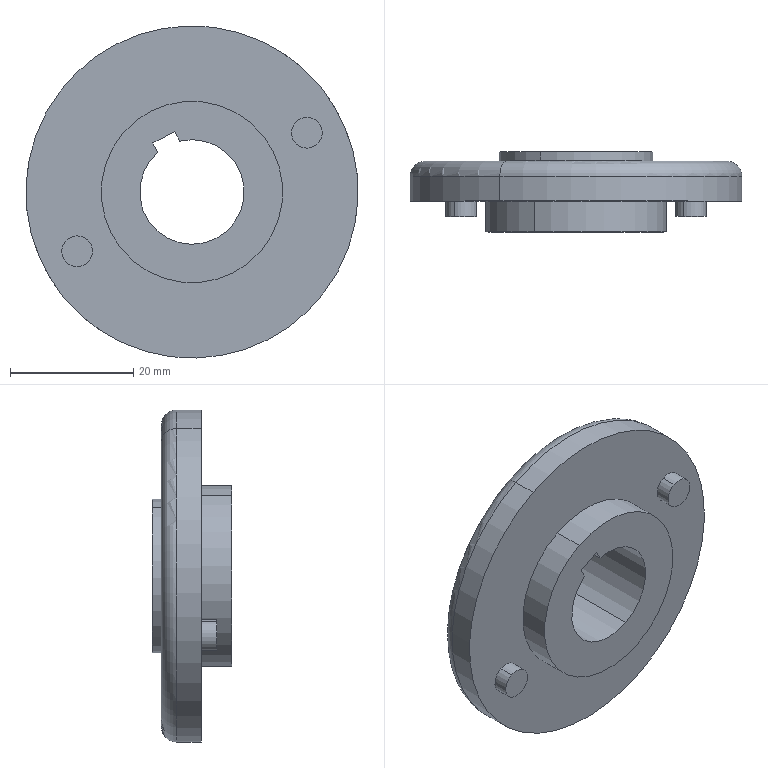Component | SolidWorks | Blade holder-1 | 1 solid | 23 faces | box 54 x 13 x 54 mm | volume 15883 mm3 | cylinder 12 | plane 9 | torus 2 | commonest cylinder face diameters 5 x4 17 x2 29.5 x2 54 x2 25 x2
build123d program:
from build123d import *

# Parameters (mm, degrees)
CONG_1_R                = 2.5
ESQUISSE3_R             = 2.5
BOSS_EXTRU_1_DEPTH      = 9
ENL_V_MAT_EXTRU_1_DEPTH = 41.336


with BuildPart() as part:
    # Esquisse1 → R_volution1 (revolve)
    with BuildSketch(Plane.XY, mode=Mode.PRIVATE) as r_volution1_sk:
        Polygon((8.5, 13), (8.5, 0), (14.75, 0), (14.75, 5), (27, 5), (27, 11.5), (12.5, 11.5), (12.5, 13), align=None)
    revolve(r_volution1_sk.sketch.rotate(Axis((0, 0, 0), (0, 1, 0)), 90), axis=Axis((0, 0, 0), (0, 1, 0)))

    # Cong_1
    cong_1_edges = [part.edges().sort_by_distance(p)[0] for p in [
        (0, 11.5, 27),
    ]]
    fillet(cong_1_edges, radius=CONG_1_R)

    # Esquisse3 → Boss.-Extru.1 (add)
    with BuildSketch(Plane(origin=(0, 11.5, 0), x_dir=(1, 0, 0), z_dir=(0, 1, 0))):
        with Locations(Location((-21, 0, 0), (0, 0, 270))):
            Circle(ESQUISSE3_R)
        with Locations(Location((21, 0, 0), (0, 0, 270))):
            Circle(ESQUISSE3_R)
    extrude(amount=-BOSS_EXTRU_1_DEPTH)

    # Esquisse4 → Enl_v. mat.-Extru.1 (cut, through all)
    with BuildSketch(Plane(origin=(0, 13, 0), x_dir=(1, 0, 0), z_dir=(0, 1, 0))):
        with BuildLine():
            Line((-2, -10), (-2, -8.261))
            ThreePointArc((-2, -8.261), (0, -8.5), (2, -8.261))
            Line((2, -8.261), (2, -10))
            Line((2, -10), (-2, -10))
        make_face()
    extrude(amount=-ENL_V_MAT_EXTRU_1_DEPTH, mode=Mode.SUBTRACT)


solid = part.part

# Placed as in the assembly
solid = solid.moved(Location((-11.038, -42.3, -47.854), (0, -27.29, 0)))
STEP:
#1=COLOUR_RGB('',0.7922,0.8196,0.9333);
#2=FILL_AREA_STYLE_COLOUR('',#1);
#3=FILL_AREA_STYLE('',(#2));
#4=SURFACE_STYLE_FILL_AREA(#3);
#5=SURFACE_SIDE_STYLE('',(#4));
#6=SURFACE_STYLE_USAGE(.BOTH.,#5);
#7=PRESENTATION_STYLE_ASSIGNMENT((#6));
#8=CARTESIAN_POINT('',(0.255,-1.567,-1.417));
#9=VERTEX_POINT('',#8);
#10=CARTESIAN_POINT('',(0.3453,-1.567,-1.592));
#11=VERTEX_POINT('',#10);
#12=CARTESIAN_POINT('',(0.3002,-1.567,-1.505));
#13=DIRECTION('',(0.,1.,-0.));
#14=DIRECTION('',(-0.4585,0.,0.8887));
#15=AXIS2_PLACEMENT_3D('',#12,#13,#14);
#16=CIRCLE('',#15,0.09843);
#17=EDGE_CURVE('',#9,#11,#16,.T.);
#18=ORIENTED_EDGE('',*,*,#17,.T.);
#19=CARTESIAN_POINT('',(0.3453,-1.469,-1.592));
#20=VERTEX_POINT('',#19);
#21=CARTESIAN_POINT('',(0.3453,-1.567,-1.592));
#22=DIRECTION('',(0.,1.,-0.));
#23=VECTOR('',#22,39.37);
#24=LINE('',#21,#23);
#25=EDGE_CURVE('',#11,#20,#24,.T.);
#26=ORIENTED_EDGE('',*,*,#25,.T.);
#27=CARTESIAN_POINT('',(0.255,-1.469,-1.417));
#28=VERTEX_POINT('',#27);
#29=CARTESIAN_POINT('',(0.3002,-1.469,-1.505));
#30=DIRECTION('',(-0.,-1.,0.));
#31=DIRECTION('',(0.4585,0.,-0.8887));
#32=AXIS2_PLACEMENT_3D('',#29,#30,#31);
#33=CIRCLE('',#32,0.09843);
#34=EDGE_CURVE('',#20,#28,#33,.T.);
#35=ORIENTED_EDGE('',*,*,#34,.T.);
#36=CARTESIAN_POINT('',(0.255,-1.567,-1.417));
#37=DIRECTION('',(0.,1.,-0.));
#38=VECTOR('',#37,39.37);
#39=LINE('',#36,#38);
#40=EDGE_CURVE('',#9,#28,#39,.T.);
#41=ORIENTED_EDGE('',*,*,#40,.F.);
#42=EDGE_LOOP('',(#18,#26,#35,#41));
#43=FACE_OUTER_BOUND('',#42,.T.);
#44=CARTESIAN_POINT('',(0.3002,-1.567,-1.505));
#45=DIRECTION('',(0.,1.,-0.));
#46=DIRECTION('',(-0.4585,0.,0.8887));
#47=AXIS2_PLACEMENT_3D('',#44,#45,#46);
#48=CYLINDRICAL_SURFACE('',#47,0.09843);
#49=ADVANCED_FACE('',(#43),#48,.T.);
#50=CARTESIAN_POINT('',(-1.214,-1.567,-2.176));
#51=VERTEX_POINT('',#50);
#52=CARTESIAN_POINT('',(-1.124,-1.567,-2.351));
#53=VERTEX_POINT('',#52);
#54=CARTESIAN_POINT('',(-1.169,-1.567,-2.263));
#55=DIRECTION('',(0.,1.,-0.));
#56=DIRECTION('',(-0.4585,0.,0.8887));
#57=AXIS2_PLACEMENT_3D('',#54,#55,#56);
#58=CIRCLE('',#57,0.09843);
#59=EDGE_CURVE('',#51,#53,#58,.T.);
#60=ORIENTED_EDGE('',*,*,#59,.T.);
#61=CARTESIAN_POINT('',(-1.124,-1.469,-2.351));
#62=VERTEX_POINT('',#61);
#63=CARTESIAN_POINT('',(-1.124,-1.567,-2.351));
#64=DIRECTION('',(0.,1.,-0.));
#65=VECTOR('',#64,39.37);
#66=LINE('',#63,#65);
#67=EDGE_CURVE('',#53,#62,#66,.T.);
#68=ORIENTED_EDGE('',*,*,#67,.T.);
#69=CARTESIAN_POINT('',(-1.214,-1.469,-2.176));
#70=VERTEX_POINT('',#69);
#71=CARTESIAN_POINT('',(-1.169,-1.469,-2.263));
#72=DIRECTION('',(-0.,-1.,0.));
#73=DIRECTION('',(0.4585,0.,-0.8887));
#74=AXIS2_PLACEMENT_3D('',#71,#72,#73);
#75=CIRCLE('',#74,0.09843);
#76=EDGE_CURVE('',#62,#70,#75,.T.);
#77=ORIENTED_EDGE('',*,*,#76,.T.);
#78=CARTESIAN_POINT('',(-1.214,-1.567,-2.176));
#79=DIRECTION('',(0.,1.,-0.));
#80=VECTOR('',#79,39.37);
#81=LINE('',#78,#80);
#82=EDGE_CURVE('',#51,#70,#81,.T.);
#83=ORIENTED_EDGE('',*,*,#82,.F.);
#84=EDGE_LOOP('',(#60,#68,#77,#83));
#85=FACE_OUTER_BOUND('',#84,.T.);
#86=CARTESIAN_POINT('',(-1.169,-1.567,-2.263));
#87=DIRECTION('',(0.,1.,-0.));
#88=DIRECTION('',(-0.4585,0.,0.8887));
#89=AXIS2_PLACEMENT_3D('',#86,#87,#88);
#90=CYLINDRICAL_SURFACE('',#89,0.09843);
#91=ADVANCED_FACE('',(#85),#90,.T.);
#92=CARTESIAN_POINT('',(0.0528,-1.311,-2.829));
#93=VERTEX_POINT('',#92);
#94=CARTESIAN_POINT('',(-0.922,-1.311,-0.9393));
#95=VERTEX_POINT('',#94);
#96=CARTESIAN_POINT('',(-0.4346,-1.311,-1.884));
#97=DIRECTION('',(-0.,-1.,0.));
#98=DIRECTION('',(-0.4585,0.,0.8887));
#99=AXIS2_PLACEMENT_3D('',#96,#97,#98);
#100=CIRCLE('',#99,1.063);
#101=EDGE_CURVE('',#93,#95,#100,.T.);
#102=ORIENTED_EDGE('',*,*,#101,.F.);
#103=CARTESIAN_POINT('',(0.007672,-1.213,-2.741));
#104=VERTEX_POINT('',#103);
#105=CARTESIAN_POINT('',(0.007672,-1.311,-2.741));
#106=DIRECTION('',(0.8887,-0.,0.4585));
#107=DIRECTION('',(0.4585,0.,-0.8887));
#108=AXIS2_PLACEMENT_3D('',#105,#106,#107);
#109=CIRCLE('',#108,0.09843);
#110=EDGE_CURVE('',#93,#104,#109,.T.);
#111=ORIENTED_EDGE('',*,*,#110,.T.);
#112=CARTESIAN_POINT('',(-0.8768,-1.213,-1.027));
#113=VERTEX_POINT('',#112);
#114=CARTESIAN_POINT('',(-0.4346,-1.213,-1.884));
#115=DIRECTION('',(0.,1.,-0.));
#116=DIRECTION('',(-0.4585,0.,0.8887));
#117=AXIS2_PLACEMENT_3D('',#114,#115,#116);
#118=CIRCLE('',#117,0.9646);
#119=EDGE_CURVE('',#113,#104,#118,.T.);
#120=ORIENTED_EDGE('',*,*,#119,.F.);
#121=CARTESIAN_POINT('',(-0.8768,-1.311,-1.027));
#122=DIRECTION('',(-0.8887,0.,-0.4585));
#123=DIRECTION('',(-0.4585,0.,0.8887));
#124=AXIS2_PLACEMENT_3D('',#121,#122,#123);
#125=CIRCLE('',#124,0.09843);
#126=EDGE_CURVE('',#95,#113,#125,.T.);
#127=ORIENTED_EDGE('',*,*,#126,.F.);
#128=EDGE_LOOP('',(#102,#111,#120,#127));
#129=FACE_OUTER_BOUND('',#128,.T.);
#130=CARTESIAN_POINT('',(-0.4346,-1.311,-1.884));
#131=DIRECTION('',(0.,1.,-0.));
#132=DIRECTION('',(-0.4585,0.,0.8887));
#133=AXIS2_PLACEMENT_3D('',#130,#131,#132);
#134=TOROIDAL_SURFACE('',#133,0.9646,0.09843);
#135=ADVANCED_FACE('',(#129),#134,.T.);
#136=CARTESIAN_POINT('',(-0.2811,-1.154,-2.181));
#137=VERTEX_POINT('',#136);
#138=CARTESIAN_POINT('',(-0.5137,-1.154,-1.559));
#139=VERTEX_POINT('',#138);
#140=CARTESIAN_POINT('',(-0.4346,-1.154,-1.884));
#141=DIRECTION('',(-0.,-1.,0.));
#142=DIRECTION('',(0.4585,-0.,-0.8887));
#143=AXIS2_PLACEMENT_3D('',#140,#141,#142);
#144=CIRCLE('',#143,0.3346);
#145=EDGE_CURVE('',#137,#139,#144,.T.);
#146=ORIENTED_EDGE('',*,*,#145,.F.);
#147=CARTESIAN_POINT('',(-0.2811,-1.665,-2.181));
#148=VERTEX_POINT('',#147);
#149=CARTESIAN_POINT('',(-0.2811,-1.665,-2.181));
#150=DIRECTION('',(-0.,-1.,0.));
#151=VECTOR('',#150,39.37);
#152=LINE('',#149,#151);
#153=EDGE_CURVE('',#137,#148,#152,.T.);
#154=ORIENTED_EDGE('',*,*,#153,.T.);
#155=CARTESIAN_POINT('',(-0.5137,-1.665,-1.559));
#156=VERTEX_POINT('',#155);
#157=CARTESIAN_POINT('',(-0.4346,-1.665,-1.884));
#158=DIRECTION('',(-0.,-1.,0.));
#159=DIRECTION('',(0.4585,-0.,-0.8887));
#160=AXIS2_PLACEMENT_3D('',#157,#158,#159);
#161=CIRCLE('',#160,0.3346);
#162=EDGE_CURVE('',#148,#156,#161,.T.);
#163=ORIENTED_EDGE('',*,*,#162,.T.);
#164=CARTESIAN_POINT('',(-0.5137,-1.665,-1.559));
#165=DIRECTION('',(0.,1.,-0.));
#166=VECTOR('',#165,39.37);
#167=LINE('',#164,#166);
#168=EDGE_CURVE('',#156,#139,#167,.T.);
#169=ORIENTED_EDGE('',*,*,#168,.T.);
#170=EDGE_LOOP('',(#146,#154,#163,#169));
#171=FACE_OUTER_BOUND('',#170,.T.);
#172=CARTESIAN_POINT('',(-0.4346,-1.665,-1.884));
#173=DIRECTION('',(-0.,-1.,0.));
#174=DIRECTION('',(0.4585,-0.,-0.8887));
#175=AXIS2_PLACEMENT_3D('',#172,#173,#174);
#176=CYLINDRICAL_SURFACE('',#175,0.3346);
#177=ADVANCED_FACE('',(#171),#176,.F.);
#178=CARTESIAN_POINT('',(-0.1683,-1.469,-2.4));
#179=VERTEX_POINT('',#178);
#180=CARTESIAN_POINT('',(-0.7008,-1.469,-1.368));
#181=VERTEX_POINT('',#180);
#182=CARTESIAN_POINT('',(-0.4346,-1.469,-1.884));
#183=DIRECTION('',(-0.,-1.,0.));
#184=DIRECTION('',(0.4585,-0.,-0.8887));
#185=AXIS2_PLACEMENT_3D('',#182,#183,#184);
#186=CIRCLE('',#185,0.5807);
#187=EDGE_CURVE('',#179,#181,#186,.T.);
#188=ORIENTED_EDGE('',*,*,#187,.T.);
#189=CARTESIAN_POINT('',(-0.7008,-1.665,-1.368));
#190=VERTEX_POINT('',#189);
#191=CARTESIAN_POINT('',(-0.7008,-1.665,-1.368));
#192=DIRECTION('',(-0.,-1.,0.));
#193=VECTOR('',#192,39.37);
#194=LINE('',#191,#193);
#195=EDGE_CURVE('',#181,#190,#194,.T.);
#196=ORIENTED_EDGE('',*,*,#195,.T.);
#197=CARTESIAN_POINT('',(-0.1683,-1.665,-2.4));
#198=VERTEX_POINT('',#197);
#199=CARTESIAN_POINT('',(-0.4346,-1.665,-1.884));
#200=DIRECTION('',(-0.,-1.,0.));
#201=DIRECTION('',(0.4585,-0.,-0.8887));
#202=AXIS2_PLACEMENT_3D('',#199,#200,#201);
#203=CIRCLE('',#202,0.5807);
#204=EDGE_CURVE('',#198,#190,#203,.T.);
#205=ORIENTED_EDGE('',*,*,#204,.F.);
#206=CARTESIAN_POINT('',(-0.1683,-1.665,-2.4));
#207=DIRECTION('',(-0.,-1.,0.));
#208=VECTOR('',#207,39.37);
#209=LINE('',#206,#208);
#210=EDGE_CURVE('',#179,#198,#209,.T.);
#211=ORIENTED_EDGE('',*,*,#210,.F.);
#212=EDGE_LOOP('',(#188,#196,#205,#211));
#213=FACE_OUTER_BOUND('',#212,.T.);
#214=CARTESIAN_POINT('',(-0.4346,-1.665,-1.884));
#215=DIRECTION('',(-0.,-1.,0.));
#216=DIRECTION('',(0.4585,-0.,-0.8887));
#217=AXIS2_PLACEMENT_3D('',#214,#215,#216);
#218=CYLINDRICAL_SURFACE('',#217,0.5807);
#219=ADVANCED_FACE('',(#213),#218,.T.);
#220=ORIENTED_EDGE('',*,*,#101,.T.);
#221=CARTESIAN_POINT('',(-0.922,-1.469,-0.9393));
#222=VERTEX_POINT('',#221);
#223=CARTESIAN_POINT('',(-0.922,-1.665,-0.9393));
#224=DIRECTION('',(-0.,-1.,0.));
#225=VECTOR('',#224,39.37);
#226=LINE('',#223,#225);
#227=EDGE_CURVE('',#95,#222,#226,.T.);
#228=ORIENTED_EDGE('',*,*,#227,.T.);
#229=CARTESIAN_POINT('',(0.0528,-1.469,-2.829));
#230=VERTEX_POINT('',#229);
#231=CARTESIAN_POINT('',(-0.4346,-1.469,-1.884));
#232=DIRECTION('',(-0.,-1.,0.));
#233=DIRECTION('',(0.4585,-0.,-0.8887));
#234=AXIS2_PLACEMENT_3D('',#231,#232,#233);
#235=CIRCLE('',#234,1.063);
#236=EDGE_CURVE('',#230,#222,#235,.T.);
#237=ORIENTED_EDGE('',*,*,#236,.F.);
#238=CARTESIAN_POINT('',(0.0528,-1.665,-2.829));
#239=DIRECTION('',(-0.,-1.,0.));
#240=VECTOR('',#239,39.37);
#241=LINE('',#238,#240);
#242=EDGE_CURVE('',#93,#230,#241,.T.);
#243=ORIENTED_EDGE('',*,*,#242,.F.);
#244=EDGE_LOOP('',(#220,#228,#237,#243));
#245=FACE_OUTER_BOUND('',#244,.T.);
#246=CARTESIAN_POINT('',(-0.4346,-1.665,-1.884));
#247=DIRECTION('',(-0.,-1.,0.));
#248=DIRECTION('',(0.4585,-0.,-0.8887));
#249=AXIS2_PLACEMENT_3D('',#246,#247,#248);
#250=CYLINDRICAL_SURFACE('',#249,1.063);
#251=ADVANCED_FACE('',(#245),#250,.T.);
#252=CARTESIAN_POINT('',(-0.2089,-1.154,-2.321));
#253=VERTEX_POINT('',#252);
#254=CARTESIAN_POINT('',(-0.6602,-1.154,-1.447));
#255=VERTEX_POINT('',#254);
#256=CARTESIAN_POINT('',(-0.4346,-1.154,-1.884));
#257=DIRECTION('',(-0.,-1.,0.));
#258=DIRECTION('',(0.4585,-0.,-0.8887));
#259=AXIS2_PLACEMENT_3D('',#256,#257,#258);
#260=CIRCLE('',#259,0.4921);
#261=EDGE_CURVE('',#253,#255,#260,.T.);
#262=ORIENTED_EDGE('',*,*,#261,.T.);
#263=CARTESIAN_POINT('',(-0.6602,-1.213,-1.447));
#264=VERTEX_POINT('',#263);
#265=CARTESIAN_POINT('',(-0.6602,-1.665,-1.447));
#266=DIRECTION('',(-0.,-1.,0.));
#267=VECTOR('',#266,39.37);
#268=LINE('',#265,#267);
#269=EDGE_CURVE('',#255,#264,#268,.T.);
#270=ORIENTED_EDGE('',*,*,#269,.T.);
#271=CARTESIAN_POINT('',(-0.2089,-1.213,-2.321));
#272=VERTEX_POINT('',#271);
#273=CARTESIAN_POINT('',(-0.4346,-1.213,-1.884));
#274=DIRECTION('',(-0.,-1.,0.));
#275=DIRECTION('',(0.4585,-0.,-0.8887));
#276=AXIS2_PLACEMENT_3D('',#273,#274,#275);
#277=CIRCLE('',#276,0.4921);
#278=EDGE_CURVE('',#272,#264,#277,.T.);
#279=ORIENTED_EDGE('',*,*,#278,.F.);
#280=CARTESIAN_POINT('',(-0.2089,-1.665,-2.321));
#281=DIRECTION('',(-0.,-1.,0.));
#282=VECTOR('',#281,39.37);
#283=LINE('',#280,#282);
#284=EDGE_CURVE('',#253,#272,#283,.T.);
#285=ORIENTED_EDGE('',*,*,#284,.F.);
#286=EDGE_LOOP('',(#262,#270,#279,#285));
#287=FACE_OUTER_BOUND('',#286,.T.);
#288=CARTESIAN_POINT('',(-0.4346,-1.665,-1.884));
#289=DIRECTION('',(-0.,-1.,0.));
#290=DIRECTION('',(0.4585,-0.,-0.8887));
#291=AXIS2_PLACEMENT_3D('',#288,#289,#290);
#292=CYLINDRICAL_SURFACE('',#291,0.4921);
#293=ADVANCED_FACE('',(#287),#292,.T.);
#294=CARTESIAN_POINT('',(-0.5451,-1.154,-1.498));
#295=VERTEX_POINT('',#294);
#296=CARTESIAN_POINT('',(-0.5451,-1.154,-1.498));
#297=DIRECTION('',(0.4585,-0.,-0.8887));
#298=VECTOR('',#297,39.37);
#299=LINE('',#296,#298);
#300=EDGE_CURVE('',#295,#139,#299,.T.);
#301=ORIENTED_EDGE('',*,*,#300,.F.);
#302=CARTESIAN_POINT('',(-0.6851,-1.154,-1.57));
#303=VERTEX_POINT('',#302);
#304=CARTESIAN_POINT('',(-0.6851,-1.154,-1.57));
#305=DIRECTION('',(0.8887,-0.,0.4585));
#306=VECTOR('',#305,39.37);
#307=LINE('',#304,#306);
#308=EDGE_CURVE('',#303,#295,#307,.T.);
#309=ORIENTED_EDGE('',*,*,#308,.F.);
#310=CARTESIAN_POINT('',(-0.6537,-1.154,-1.631));
#311=VERTEX_POINT('',#310);
#312=CARTESIAN_POINT('',(-0.6851,-1.154,-1.57));
#313=DIRECTION('',(-0.4585,0.,0.8887));
#314=VECTOR('',#313,39.37);
#315=LINE('',#312,#314);
#316=EDGE_CURVE('',#311,#303,#315,.T.);
#317=ORIENTED_EDGE('',*,*,#316,.F.);
#318=CARTESIAN_POINT('',(-0.4346,-1.154,-1.884));
#319=DIRECTION('',(-0.,-1.,0.));
#320=DIRECTION('',(0.4585,-0.,-0.8887));
#321=AXIS2_PLACEMENT_3D('',#318,#319,#320);
#322=CIRCLE('',#321,0.3346);
#323=EDGE_CURVE('',#311,#137,#322,.T.);
#324=ORIENTED_EDGE('',*,*,#323,.T.);
#325=ORIENTED_EDGE('',*,*,#145,.T.);
#326=EDGE_LOOP('',(#301,#309,#317,#324,#325));
#327=FACE_BOUND('',#326,.T.);
#328=ORIENTED_EDGE('',*,*,#261,.F.);
#329=CARTESIAN_POINT('',(-0.4346,-1.154,-1.884));
#330=DIRECTION('',(-0.,-1.,0.));
#331=DIRECTION('',(0.4585,-0.,-0.8887));
#332=AXIS2_PLACEMENT_3D('',#329,#330,#331);
#333=CIRCLE('',#332,0.4921);
#334=EDGE_CURVE('',#255,#253,#333,.T.);
#335=ORIENTED_EDGE('',*,*,#334,.F.);
#336=EDGE_LOOP('',(#328,#335));
#337=FACE_OUTER_BOUND('',#336,.T.);
#338=CARTESIAN_POINT('',(-0.1372,-1.154,-1.731));
#339=DIRECTION('',(0.,1.,-0.));
#340=DIRECTION('',(-0.4585,0.,0.8887));
#341=AXIS2_PLACEMENT_3D('',#338,#339,#340);
#342=PLANE('',#341);
#343=ADVANCED_FACE('',(#327,#337),#342,.T.);
#344=ORIENTED_EDGE('',*,*,#269,.F.);
#345=ORIENTED_EDGE('',*,*,#334,.T.);
#346=ORIENTED_EDGE('',*,*,#284,.T.);
#347=CARTESIAN_POINT('',(-0.4346,-1.213,-1.884));
#348=DIRECTION('',(-0.,-1.,0.));
#349=DIRECTION('',(0.4585,-0.,-0.8887));
#350=AXIS2_PLACEMENT_3D('',#347,#348,#349);
#351=CIRCLE('',#350,0.4921);
#352=EDGE_CURVE('',#264,#272,#351,.T.);
#353=ORIENTED_EDGE('',*,*,#352,.F.);
#354=EDGE_LOOP('',(#344,#345,#346,#353));
#355=FACE_OUTER_BOUND('',#354,.T.);
#356=CARTESIAN_POINT('',(-0.4346,-1.665,-1.884));
#357=DIRECTION('',(-0.,-1.,0.));
#358=DIRECTION('',(0.4585,-0.,-0.8887));
#359=AXIS2_PLACEMENT_3D('',#356,#357,#358);
#360=CYLINDRICAL_SURFACE('',#359,0.4921);
#361=ADVANCED_FACE('',(#355),#360,.T.);
#362=ORIENTED_EDGE('',*,*,#119,.T.);
#363=CARTESIAN_POINT('',(-0.4346,-1.213,-1.884));
#364=DIRECTION('',(0.,1.,-0.));
#365=DIRECTION('',(-0.4585,0.,0.8887));
#366=AXIS2_PLACEMENT_3D('',#363,#364,#365);
#367=CIRCLE('',#366,0.9646);
#368=EDGE_CURVE('',#104,#113,#367,.T.);
#369=ORIENTED_EDGE('',*,*,#368,.T.);
#370=EDGE_LOOP('',(#362,#369));
#371=FACE_OUTER_BOUND('',#370,.T.);
#372=ORIENTED_EDGE('',*,*,#278,.T.);
#373=ORIENTED_EDGE('',*,*,#352,.T.);
#374=EDGE_LOOP('',(#372,#373));
#375=FACE_BOUND('',#374,.T.);
#376=CARTESIAN_POINT('',(0.5101,-1.213,-1.397));
#377=DIRECTION('',(0.,1.,-0.));
#378=DIRECTION('',(-0.4585,0.,0.8887));
#379=AXIS2_PLACEMENT_3D('',#376,#377,#378);
#380=PLANE('',#379);
#381=ADVANCED_FACE('',(#371,#375),#380,.T.);
#382=ORIENTED_EDGE('',*,*,#227,.F.);
#383=CARTESIAN_POINT('',(-0.4346,-1.311,-1.884));
#384=DIRECTION('',(-0.,-1.,0.));
#385=DIRECTION('',(-0.4585,0.,0.8887));
#386=AXIS2_PLACEMENT_3D('',#383,#384,#385);
#387=CIRCLE('',#386,1.063);
#388=EDGE_CURVE('',#95,#93,#387,.T.);
#389=ORIENTED_EDGE('',*,*,#388,.T.);
#390=ORIENTED_EDGE('',*,*,#242,.T.);
#391=CARTESIAN_POINT('',(-0.4346,-1.469,-1.884));
#392=DIRECTION('',(-0.,-1.,0.));
#393=DIRECTION('',(0.4585,-0.,-0.8887));
#394=AXIS2_PLACEMENT_3D('',#391,#392,#393);
#395=CIRCLE('',#394,1.063);
#396=EDGE_CURVE('',#222,#230,#395,.T.);
#397=ORIENTED_EDGE('',*,*,#396,.F.);
#398=EDGE_LOOP('',(#382,#389,#390,#397));
#399=FACE_OUTER_BOUND('',#398,.T.);
#400=CARTESIAN_POINT('',(-0.4346,-1.665,-1.884));
#401=DIRECTION('',(-0.,-1.,0.));
#402=DIRECTION('',(0.4585,-0.,-0.8887));
#403=AXIS2_PLACEMENT_3D('',#400,#401,#402);
#404=CYLINDRICAL_SURFACE('',#403,1.063);
#405=ADVANCED_FACE('',(#399),#404,.T.);
#406=CARTESIAN_POINT('',(0.3002,-1.469,-1.505));
#407=DIRECTION('',(-0.,-1.,0.));
#408=DIRECTION('',(0.4585,0.,-0.8887));
#409=AXIS2_PLACEMENT_3D('',#406,#407,#408);
#410=CIRCLE('',#409,0.09843);
#411=EDGE_CURVE('',#28,#20,#410,.T.);
#412=ORIENTED_EDGE('',*,*,#411,.F.);
#413=ORIENTED_EDGE('',*,*,#34,.F.);
#414=EDGE_LOOP('',(#412,#413));
#415=FACE_BOUND('',#414,.T.);
#416=CARTESIAN_POINT('',(-1.169,-1.469,-2.263));
#417=DIRECTION('',(-0.,-1.,0.));
#418=DIRECTION('',(0.4585,0.,-0.8887));
#419=AXIS2_PLACEMENT_3D('',#416,#417,#418);
#420=CIRCLE('',#419,0.09843);
#421=EDGE_CURVE('',#70,#62,#420,.T.);
#422=ORIENTED_EDGE('',*,*,#421,.F.);
#423=ORIENTED_EDGE('',*,*,#76,.F.);
#424=EDGE_LOOP('',(#422,#423));
#425=FACE_BOUND('',#424,.T.);
#426=ORIENTED_EDGE('',*,*,#236,.T.);
#427=ORIENTED_EDGE('',*,*,#396,.T.);
#428=EDGE_LOOP('',(#426,#427));
#429=FACE_OUTER_BOUND('',#428,.T.);
#430=ORIENTED_EDGE('',*,*,#187,.F.);
#431=CARTESIAN_POINT('',(-0.4346,-1.469,-1.884));
#432=DIRECTION('',(-0.,-1.,0.));
#433=DIRECTION('',(0.4585,-0.,-0.8887));
#434=AXIS2_PLACEMENT_3D('',#431,#432,#433);
#435=CIRCLE('',#434,0.5807);
#436=EDGE_CURVE('',#181,#179,#435,.T.);
#437=ORIENTED_EDGE('',*,*,#436,.F.);
#438=EDGE_LOOP('',(#430,#437));
#439=FACE_BOUND('',#438,.T.);
#440=CARTESIAN_POINT('',(0.08149,-1.469,-1.618));
#441=DIRECTION('',(-0.,-1.,0.));
#442=DIRECTION('',(0.4585,-0.,-0.8887));
#443=AXIS2_PLACEMENT_3D('',#440,#441,#442);
#444=PLANE('',#443);
#445=ADVANCED_FACE('',(#415,#425,#429,#439),#444,.T.);
#446=ORIENTED_EDGE('',*,*,#195,.F.);
#447=ORIENTED_EDGE('',*,*,#436,.T.);
#448=ORIENTED_EDGE('',*,*,#210,.T.);
#449=CARTESIAN_POINT('',(-0.4346,-1.665,-1.884));
#450=DIRECTION('',(-0.,-1.,0.));
#451=DIRECTION('',(0.4585,-0.,-0.8887));
#452=AXIS2_PLACEMENT_3D('',#449,#450,#451);
#453=CIRCLE('',#452,0.5807);
#454=EDGE_CURVE('',#190,#198,#453,.T.);
#455=ORIENTED_EDGE('',*,*,#454,.F.);
#456=EDGE_LOOP('',(#446,#447,#448,#455));
#457=FACE_OUTER_BOUND('',#456,.T.);
#458=CARTESIAN_POINT('',(-0.4346,-1.665,-1.884));
#459=DIRECTION('',(-0.,-1.,0.));
#460=DIRECTION('',(0.4585,-0.,-0.8887));
#461=AXIS2_PLACEMENT_3D('',#458,#459,#460);
#462=CYLINDRICAL_SURFACE('',#461,0.5807);
#463=ADVANCED_FACE('',(#457),#462,.T.);
#464=CARTESIAN_POINT('',(-0.5451,-1.665,-1.498));
#465=VERTEX_POINT('',#464);
#466=CARTESIAN_POINT('',(-0.5451,-1.665,-1.498));
#467=DIRECTION('',(0.4585,-0.,-0.8887));
#468=VECTOR('',#467,39.37);
#469=LINE('',#466,#468);
#470=EDGE_CURVE('',#465,#156,#469,.T.);
#471=ORIENTED_EDGE('',*,*,#470,.T.);
#472=ORIENTED_EDGE('',*,*,#162,.F.);
#473=CARTESIAN_POINT('',(-0.6537,-1.665,-1.631));
#474=VERTEX_POINT('',#473);
#475=CARTESIAN_POINT('',(-0.4346,-1.665,-1.884));
#476=DIRECTION('',(-0.,-1.,0.));
#477=DIRECTION('',(0.4585,-0.,-0.8887));
#478=AXIS2_PLACEMENT_3D('',#475,#476,#477);
#479=CIRCLE('',#478,0.3346);
#480=EDGE_CURVE('',#474,#148,#479,.T.);
#481=ORIENTED_EDGE('',*,*,#480,.F.);
#482=CARTESIAN_POINT('',(-0.6851,-1.665,-1.57));
#483=VERTEX_POINT('',#482);
#484=CARTESIAN_POINT('',(-0.6851,-1.665,-1.57));
#485=DIRECTION('',(-0.4585,0.,0.8887));
#486=VECTOR('',#485,39.37);
#487=LINE('',#484,#486);
#488=EDGE_CURVE('',#474,#483,#487,.T.);
#489=ORIENTED_EDGE('',*,*,#488,.T.);
#490=CARTESIAN_POINT('',(-0.6851,-1.665,-1.57));
#491=DIRECTION('',(0.8887,-0.,0.4585));
#492=VECTOR('',#491,39.37);
#493=LINE('',#490,#492);
#494=EDGE_CURVE('',#483,#465,#493,.T.);
#495=ORIENTED_EDGE('',*,*,#494,.T.);
#496=EDGE_LOOP('',(#471,#472,#481,#489,#495));
#497=FACE_BOUND('',#496,.T.);
#498=ORIENTED_EDGE('',*,*,#204,.T.);
#499=ORIENTED_EDGE('',*,*,#454,.T.);
#500=EDGE_LOOP('',(#498,#499));
#501=FACE_OUTER_BOUND('',#500,.T.);
#502=CARTESIAN_POINT('',(-0.1372,-1.665,-1.731));
#503=DIRECTION('',(-0.,-1.,0.));
#504=DIRECTION('',(0.4585,-0.,-0.8887));
#505=AXIS2_PLACEMENT_3D('',#502,#503,#504);
#506=PLANE('',#505);
#507=ADVANCED_FACE('',(#497,#501),#506,.T.);
#508=ORIENTED_EDGE('',*,*,#153,.F.);
#509=ORIENTED_EDGE('',*,*,#323,.F.);
#510=CARTESIAN_POINT('',(-0.6537,-1.665,-1.631));
#511=DIRECTION('',(0.,1.,-0.));
#512=VECTOR('',#511,39.37);
#513=LINE('',#510,#512);
#514=EDGE_CURVE('',#474,#311,#513,.T.);
#515=ORIENTED_EDGE('',*,*,#514,.F.);
#516=ORIENTED_EDGE('',*,*,#480,.T.);
#517=EDGE_LOOP('',(#508,#509,#515,#516));
#518=FACE_OUTER_BOUND('',#517,.T.);
#519=CARTESIAN_POINT('',(-0.4346,-1.665,-1.884));
#520=DIRECTION('',(-0.,-1.,0.));
#521=DIRECTION('',(0.4585,-0.,-0.8887));
#522=AXIS2_PLACEMENT_3D('',#519,#520,#521);
#523=CYLINDRICAL_SURFACE('',#522,0.3346);
#524=ADVANCED_FACE('',(#518),#523,.F.);
#525=ORIENTED_EDGE('',*,*,#110,.F.);
#526=ORIENTED_EDGE('',*,*,#388,.F.);
#527=ORIENTED_EDGE('',*,*,#126,.T.);
#528=ORIENTED_EDGE('',*,*,#368,.F.);
#529=EDGE_LOOP('',(#525,#526,#527,#528));
#530=FACE_OUTER_BOUND('',#529,.T.);
#531=CARTESIAN_POINT('',(-0.4346,-1.311,-1.884));
#532=DIRECTION('',(0.,1.,-0.));
#533=DIRECTION('',(-0.4585,0.,0.8887));
#534=AXIS2_PLACEMENT_3D('',#531,#532,#533);
#535=TOROIDAL_SURFACE('',#534,0.9646,0.09843);
#536=ADVANCED_FACE('',(#530),#535,.T.);
#537=ORIENTED_EDGE('',*,*,#67,.F.);
#538=CARTESIAN_POINT('',(-1.169,-1.567,-2.263));
#539=DIRECTION('',(0.,1.,-0.));
#540=DIRECTION('',(-0.4585,0.,0.8887));
#541=AXIS2_PLACEMENT_3D('',#538,#539,#540);
#542=CIRCLE('',#541,0.09843);
#543=EDGE_CURVE('',#53,#51,#542,.T.);
#544=ORIENTED_EDGE('',*,*,#543,.T.);
#545=ORIENTED_EDGE('',*,*,#82,.T.);
#546=ORIENTED_EDGE('',*,*,#421,.T.);
#547=EDGE_LOOP('',(#537,#544,#545,#546));
#548=FACE_OUTER_BOUND('',#547,.T.);
#549=CARTESIAN_POINT('',(-1.169,-1.567,-2.263));
#550=DIRECTION('',(0.,1.,-0.));
#551=DIRECTION('',(-0.4585,0.,0.8887));
#552=AXIS2_PLACEMENT_3D('',#549,#550,#551);
#553=CYLINDRICAL_SURFACE('',#552,0.09843);
#554=ADVANCED_FACE('',(#548),#553,.T.);
#555=ORIENTED_EDGE('',*,*,#59,.F.);
#556=ORIENTED_EDGE('',*,*,#543,.F.);
#557=EDGE_LOOP('',(#555,#556));
#558=FACE_OUTER_BOUND('',#557,.T.);
#559=CARTESIAN_POINT('',(-1.169,-1.567,-2.263));
#560=DIRECTION('',(0.,1.,-0.));
#561=DIRECTION('',(-0.4585,0.,0.8887));
#562=AXIS2_PLACEMENT_3D('',#559,#560,#561);
#563=PLANE('',#562);
#564=ADVANCED_FACE('',(#558),#563,.F.);
#565=ORIENTED_EDGE('',*,*,#25,.F.);
#566=CARTESIAN_POINT('',(0.3002,-1.567,-1.505));
#567=DIRECTION('',(0.,1.,-0.));
#568=DIRECTION('',(-0.4585,0.,0.8887));
#569=AXIS2_PLACEMENT_3D('',#566,#567,#568);
#570=CIRCLE('',#569,0.09843);
#571=EDGE_CURVE('',#11,#9,#570,.T.);
#572=ORIENTED_EDGE('',*,*,#571,.T.);
#573=ORIENTED_EDGE('',*,*,#40,.T.);
#574=ORIENTED_EDGE('',*,*,#411,.T.);
#575=EDGE_LOOP('',(#565,#572,#573,#574));
#576=FACE_OUTER_BOUND('',#575,.T.);
#577=CARTESIAN_POINT('',(0.3002,-1.567,-1.505));
#578=DIRECTION('',(0.,1.,-0.));
#579=DIRECTION('',(-0.4585,0.,0.8887));
#580=AXIS2_PLACEMENT_3D('',#577,#578,#579);
#581=CYLINDRICAL_SURFACE('',#580,0.09843);
#582=ADVANCED_FACE('',(#576),#581,.T.);
#583=ORIENTED_EDGE('',*,*,#17,.F.);
#584=ORIENTED_EDGE('',*,*,#571,.F.);
#585=EDGE_LOOP('',(#583,#584));
#586=FACE_OUTER_BOUND('',#585,.T.);
#587=CARTESIAN_POINT('',(0.3002,-1.567,-1.505));
#588=DIRECTION('',(0.,1.,-0.));
#589=DIRECTION('',(-0.4585,0.,0.8887));
#590=AXIS2_PLACEMENT_3D('',#587,#588,#589);
#591=PLANE('',#590);
#592=ADVANCED_FACE('',(#586),#591,.F.);
#593=ORIENTED_EDGE('',*,*,#300,.T.);
#594=ORIENTED_EDGE('',*,*,#168,.F.);
#595=ORIENTED_EDGE('',*,*,#470,.F.);
#596=CARTESIAN_POINT('',(-0.5451,-1.665,-1.498));
#597=DIRECTION('',(0.,1.,-0.));
#598=VECTOR('',#597,39.37);
#599=LINE('',#596,#598);
#600=EDGE_CURVE('',#465,#295,#599,.T.);
#601=ORIENTED_EDGE('',*,*,#600,.T.);
#602=EDGE_LOOP('',(#593,#594,#595,#601));
#603=FACE_OUTER_BOUND('',#602,.T.);
#604=CARTESIAN_POINT('',(-0.5451,-1.665,-1.498));
#605=DIRECTION('',(0.8887,-0.,0.4585));
#606=DIRECTION('',(0.4585,-0.,-0.8887));
#607=AXIS2_PLACEMENT_3D('',#604,#605,#606);
#608=PLANE('',#607);
#609=ADVANCED_FACE('',(#603),#608,.F.);
#610=ORIENTED_EDGE('',*,*,#308,.T.);
#611=ORIENTED_EDGE('',*,*,#600,.F.);
#612=ORIENTED_EDGE('',*,*,#494,.F.);
#613=CARTESIAN_POINT('',(-0.6851,-1.665,-1.57));
#614=DIRECTION('',(0.,1.,-0.));
#615=VECTOR('',#614,39.37);
#616=LINE('',#613,#615);
#617=EDGE_CURVE('',#483,#303,#616,.T.);
#618=ORIENTED_EDGE('',*,*,#617,.T.);
#619=EDGE_LOOP('',(#610,#611,#612,#618));
#620=FACE_OUTER_BOUND('',#619,.T.);
#621=CARTESIAN_POINT('',(-0.6851,-1.665,-1.57));
#622=DIRECTION('',(-0.4585,0.,0.8887));
#623=DIRECTION('',(0.8887,-0.,0.4585));
#624=AXIS2_PLACEMENT_3D('',#621,#622,#623);
#625=PLANE('',#624);
#626=ADVANCED_FACE('',(#620),#625,.F.);
#627=ORIENTED_EDGE('',*,*,#316,.T.);
#628=ORIENTED_EDGE('',*,*,#617,.F.);
#629=ORIENTED_EDGE('',*,*,#488,.F.);
#630=ORIENTED_EDGE('',*,*,#514,.T.);
#631=EDGE_LOOP('',(#627,#628,#629,#630));
#632=FACE_OUTER_BOUND('',#631,.T.);
#633=CARTESIAN_POINT('',(-0.6851,-1.665,-1.57));
#634=DIRECTION('',(-0.8887,0.,-0.4585));
#635=DIRECTION('',(-0.4585,0.,0.8887));
#636=AXIS2_PLACEMENT_3D('',#633,#634,#635);
#637=PLANE('',#636);
#638=ADVANCED_FACE('',(#632),#637,.F.);
#639=CLOSED_SHELL('',(#49,#91,#135,#177,#219,#251,#293,#343,#361,#381,#405,#445,#463,#507,#524,#536,#554,#564,#582,#592,#609,#626,#638));
#640=MANIFOLD_SOLID_BREP('',#639);
#641=STYLED_ITEM('',(#7),#640);
#642=PRESENTATION_LAYER_ASSIGNMENT('','',(#641));
#643=CARTESIAN_POINT('',(0.,0.,0.));
#644=DIRECTION('',(0.,0.,1.));
#645=DIRECTION('',(1.,0.,0.));
#646=AXIS2_PLACEMENT_3D('',#643,#644,#645);
#647=(LENGTH_UNIT()NAMED_UNIT(*)SI_UNIT($,.METRE.));
#648=LENGTH_MEASURE_WITH_UNIT(LENGTH_MEASURE(0.0254),#647);
#649=DIMENSIONAL_EXPONENTS(1.,0.,0.,0.,0.,0.,0.);
#650=(CONVERSION_BASED_UNIT('',#648)LENGTH_UNIT()NAMED_UNIT(#649));
#651=UNCERTAINTY_MEASURE_WITH_UNIT(LENGTH_MEASURE(0.00001),#650,'','');
#652=(NAMED_UNIT(*)PLANE_ANGLE_UNIT()SI_UNIT($,.RADIAN.));
#653=(NAMED_UNIT(*)SI_UNIT($,.STERADIAN.)SOLID_ANGLE_UNIT());
#654=(GEOMETRIC_REPRESENTATION_CONTEXT(3)GLOBAL_UNCERTAINTY_ASSIGNED_CONTEXT((#651))GLOBAL_UNIT_ASSIGNED_CONTEXT((#650,#652,#653))REPRESENTATION_CONTEXT('',''));
#655=ADVANCED_BREP_SHAPE_REPRESENTATION('',(#640,#646),#654);
#656=(LENGTH_UNIT()NAMED_UNIT(*)SI_UNIT($,.METRE.));
#657=LENGTH_MEASURE_WITH_UNIT(LENGTH_MEASURE(0.0254),#656);
#658=DIMENSIONAL_EXPONENTS(1.,0.,0.,0.,0.,0.,0.);
#659=(CONVERSION_BASED_UNIT('',#657)LENGTH_UNIT()NAMED_UNIT(#658));
#660=UNCERTAINTY_MEASURE_WITH_UNIT(LENGTH_MEASURE(0.00001),#659,'','');
#661=(NAMED_UNIT(*)PLANE_ANGLE_UNIT()SI_UNIT($,.RADIAN.));
#662=(NAMED_UNIT(*)SI_UNIT($,.STERADIAN.)SOLID_ANGLE_UNIT());
#663=(GEOMETRIC_REPRESENTATION_CONTEXT(3)GLOBAL_UNCERTAINTY_ASSIGNED_CONTEXT((#660))GLOBAL_UNIT_ASSIGNED_CONTEXT((#659,#661,#662))REPRESENTATION_CONTEXT('',''));
#664=MECHANICAL_DESIGN_GEOMETRIC_PRESENTATION_REPRESENTATION('',(#641),#663);